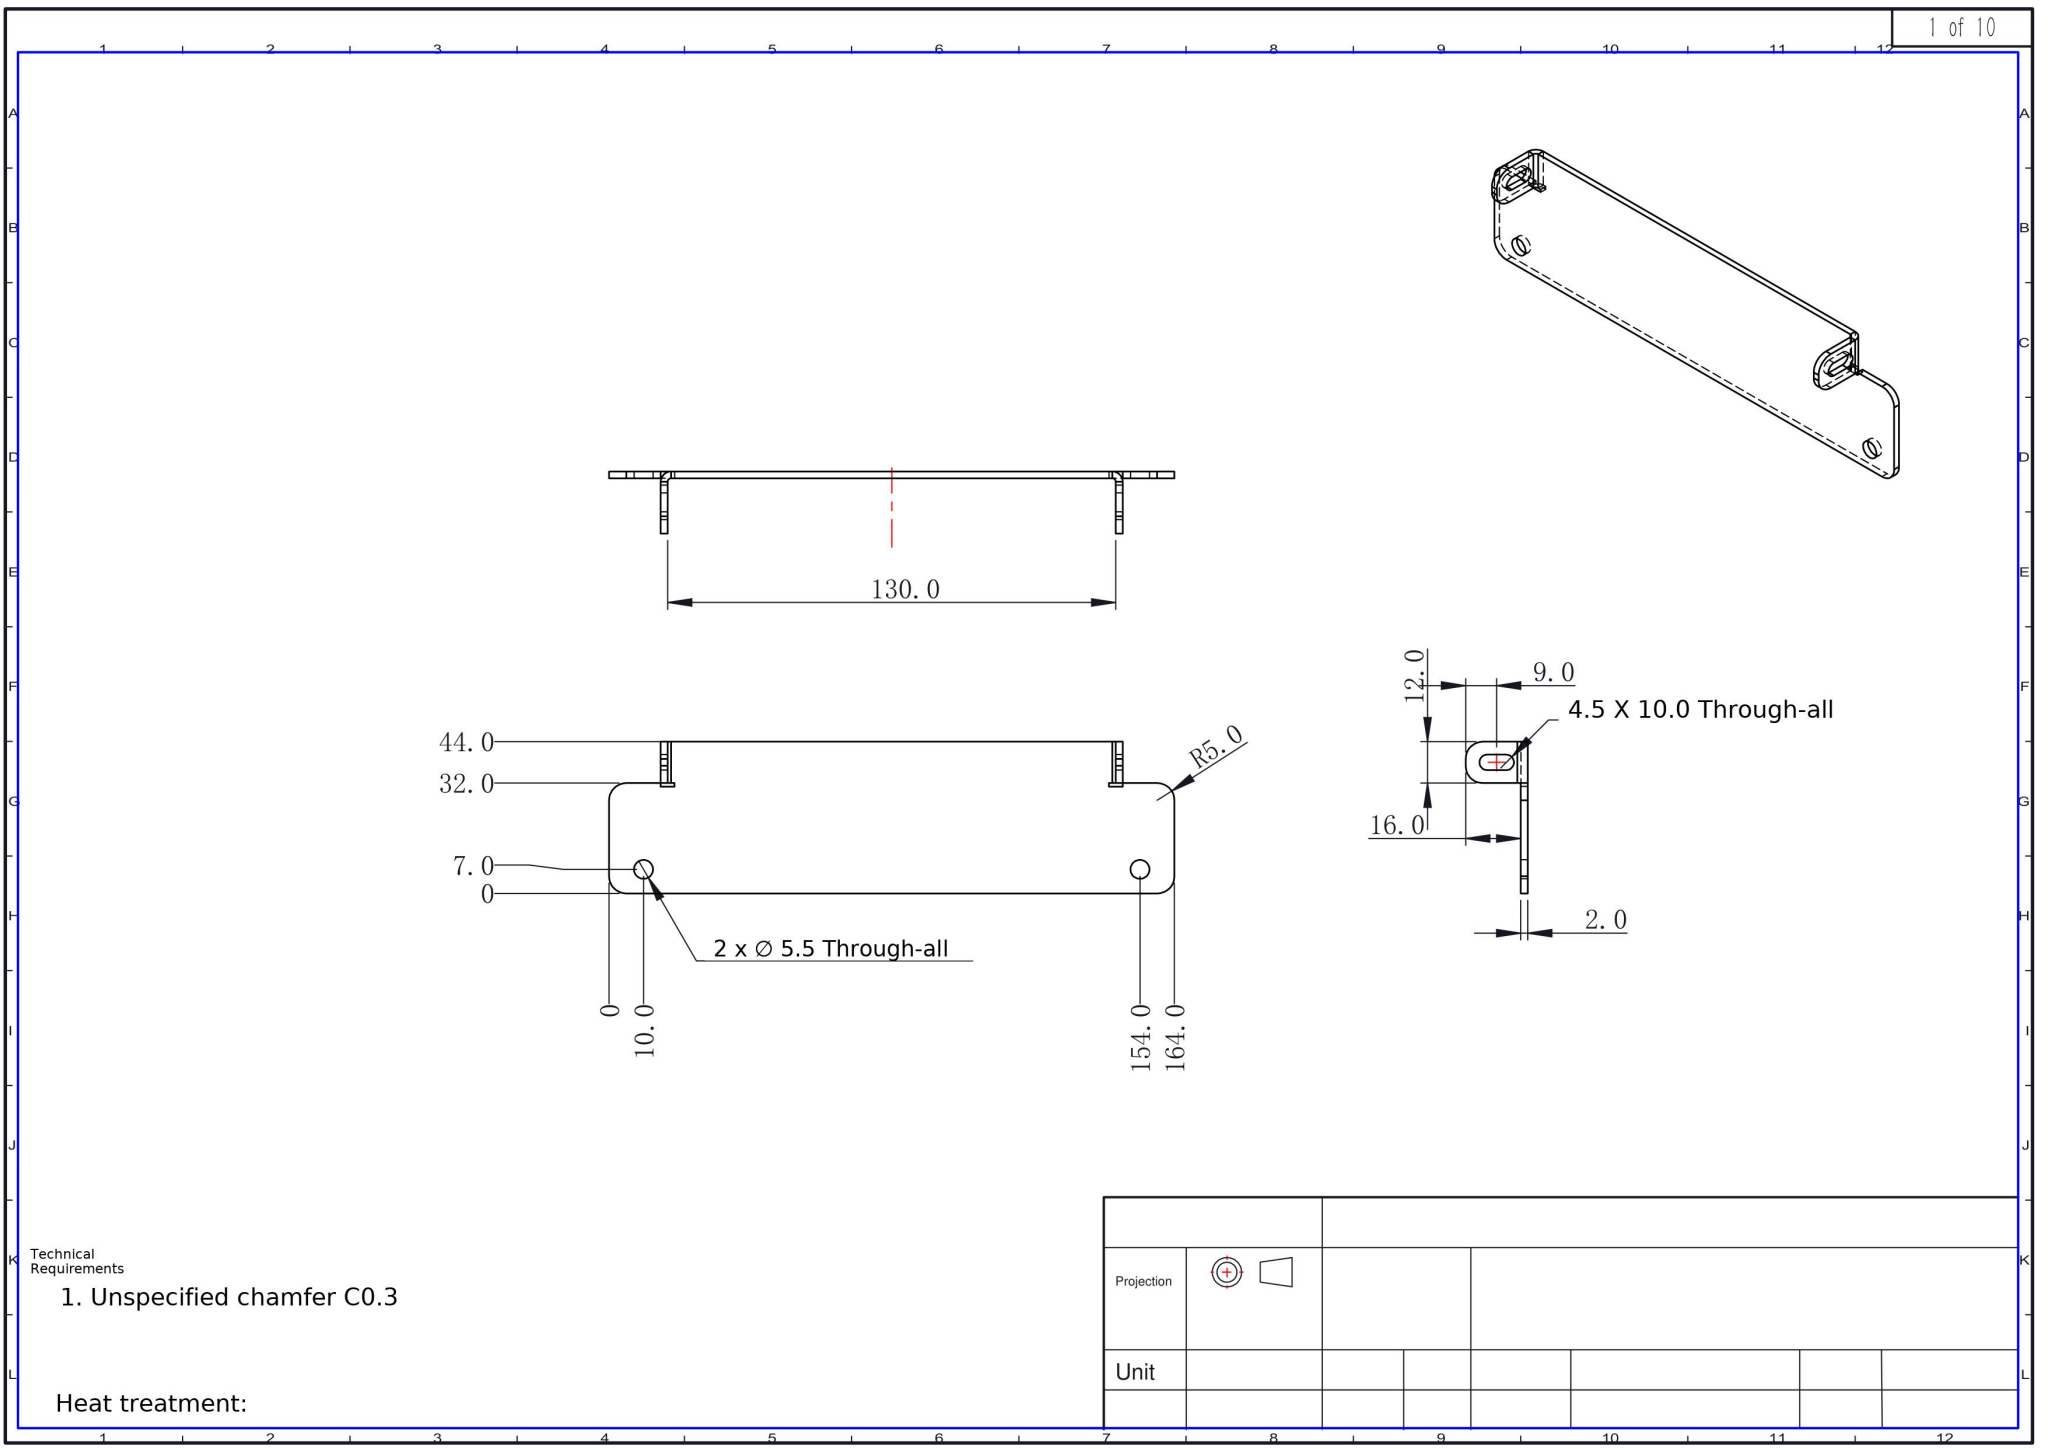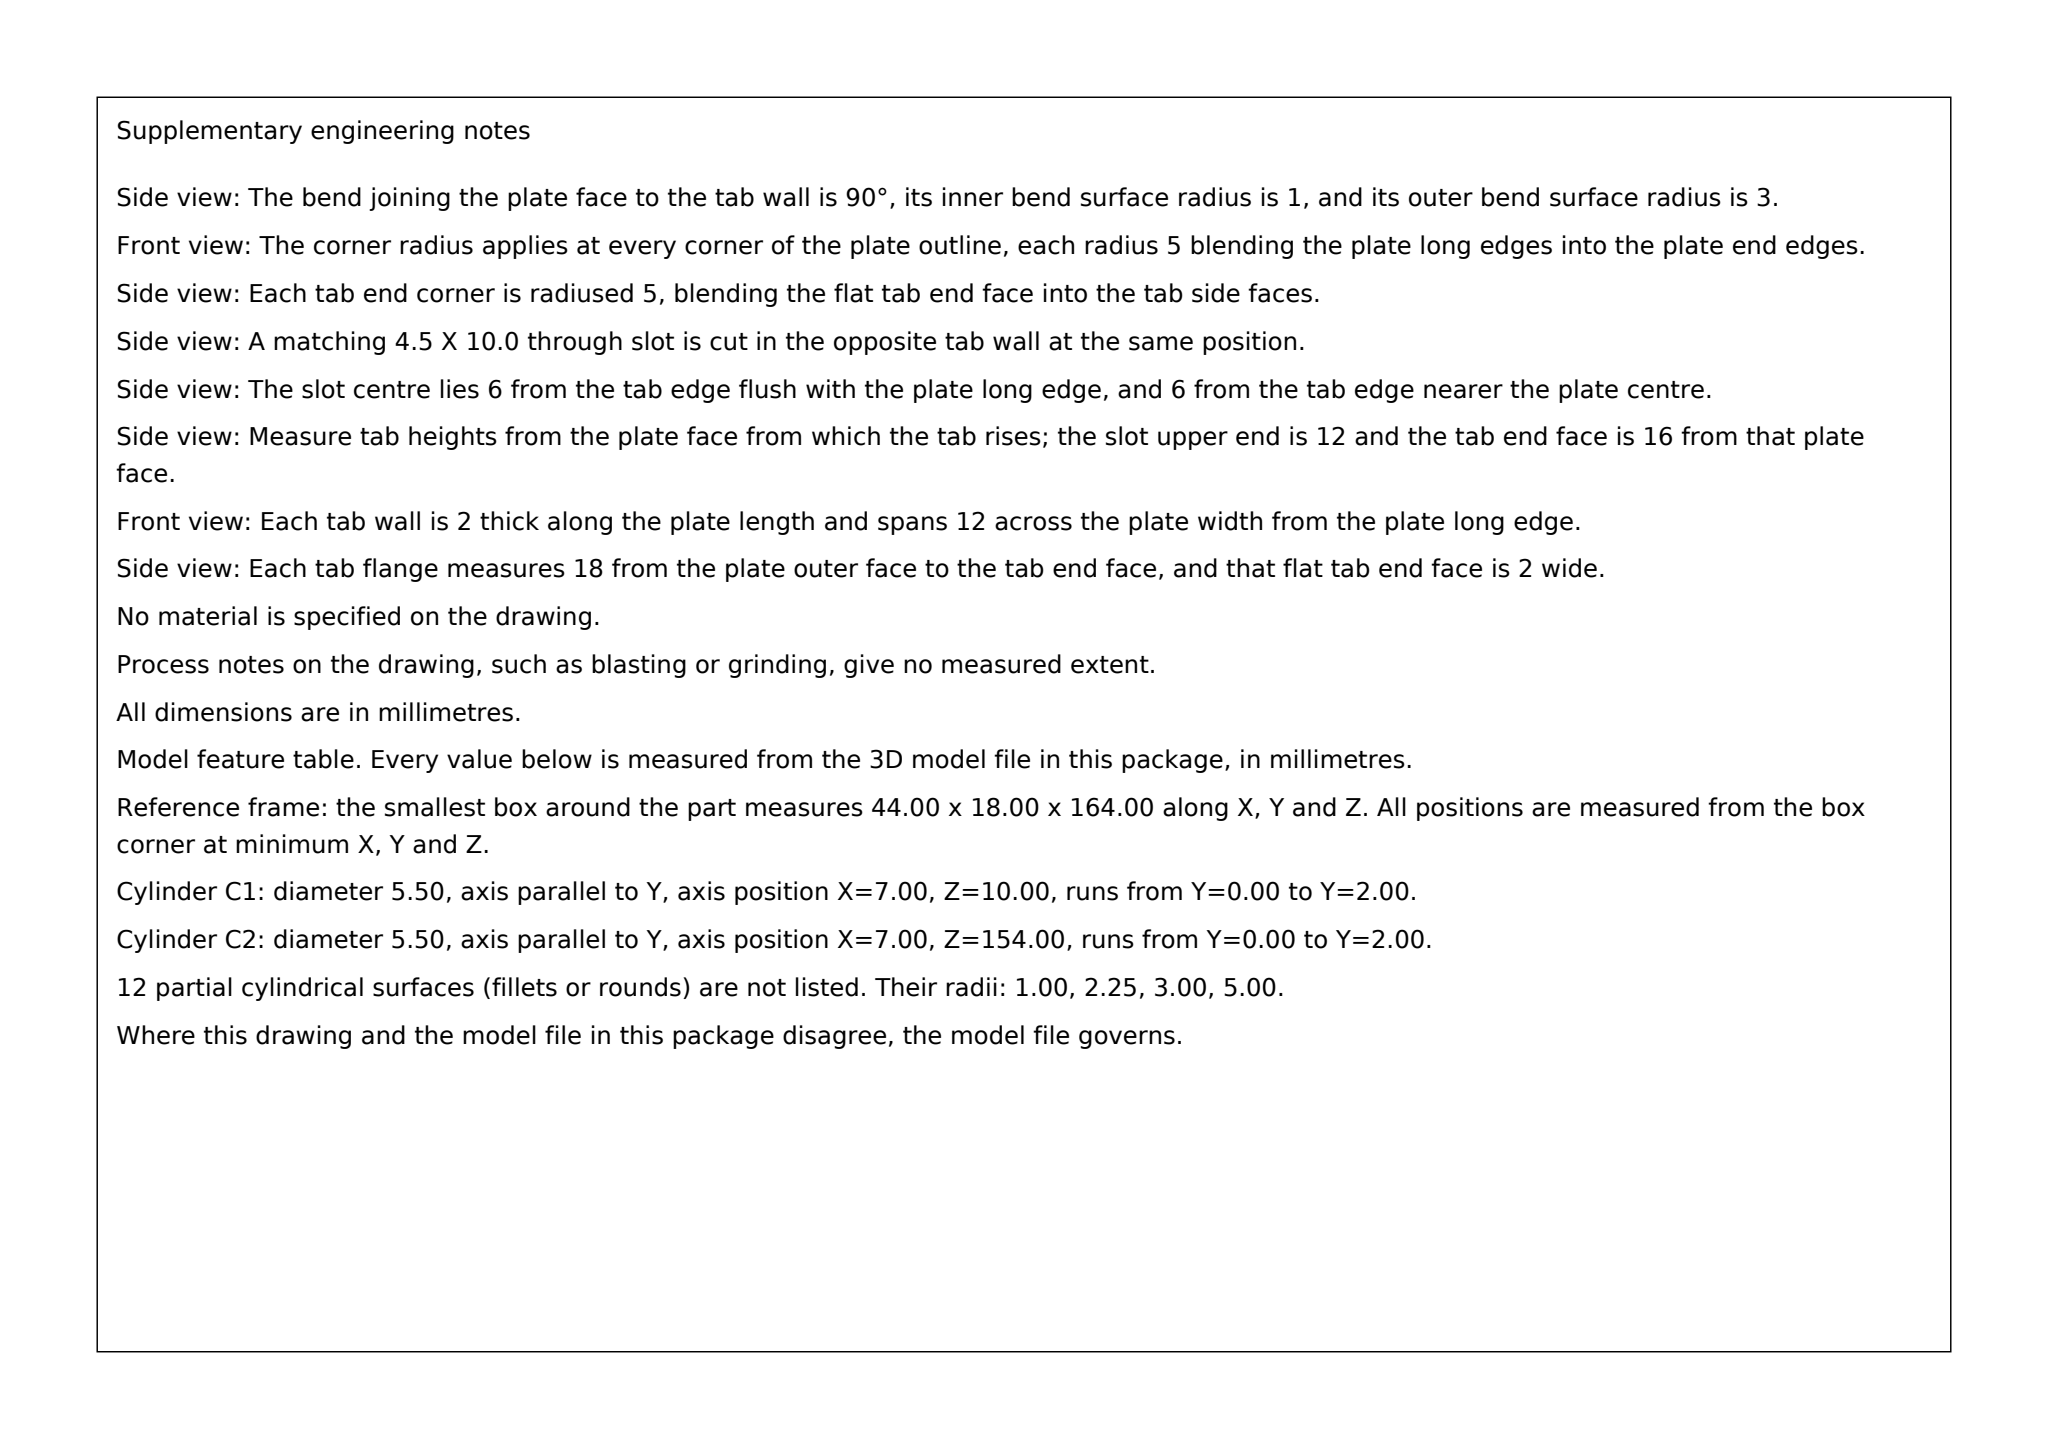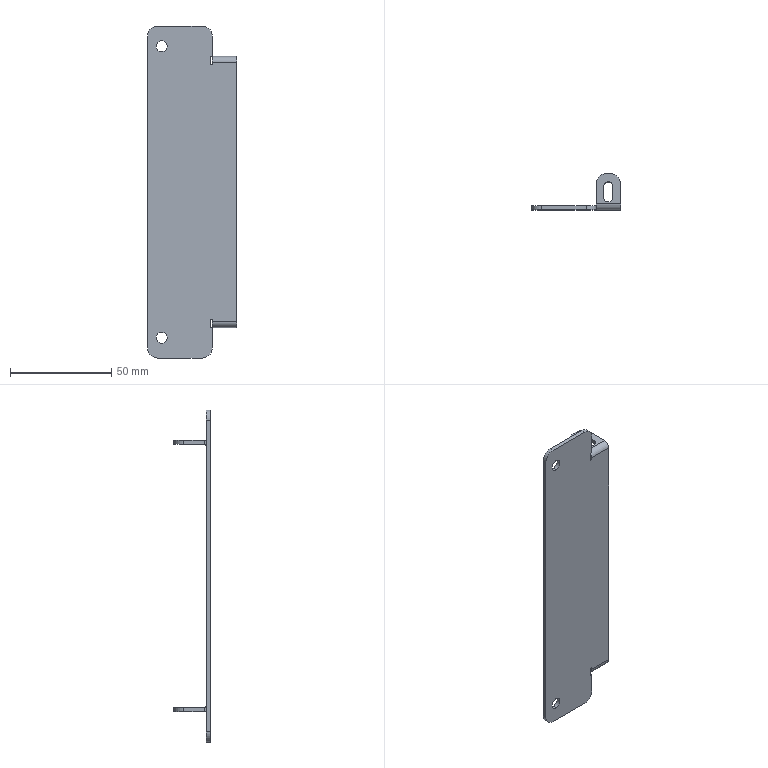Part | SolidWorks | mm | 1 solid | 56 faces | box 44 x 18 x 164 mm | volume 14079 mm3 | plane 34 | cylinder 22 | commonest cylinder face diameters 10 x8 4.5 x6 5.5 x4 6 x2 2 x2